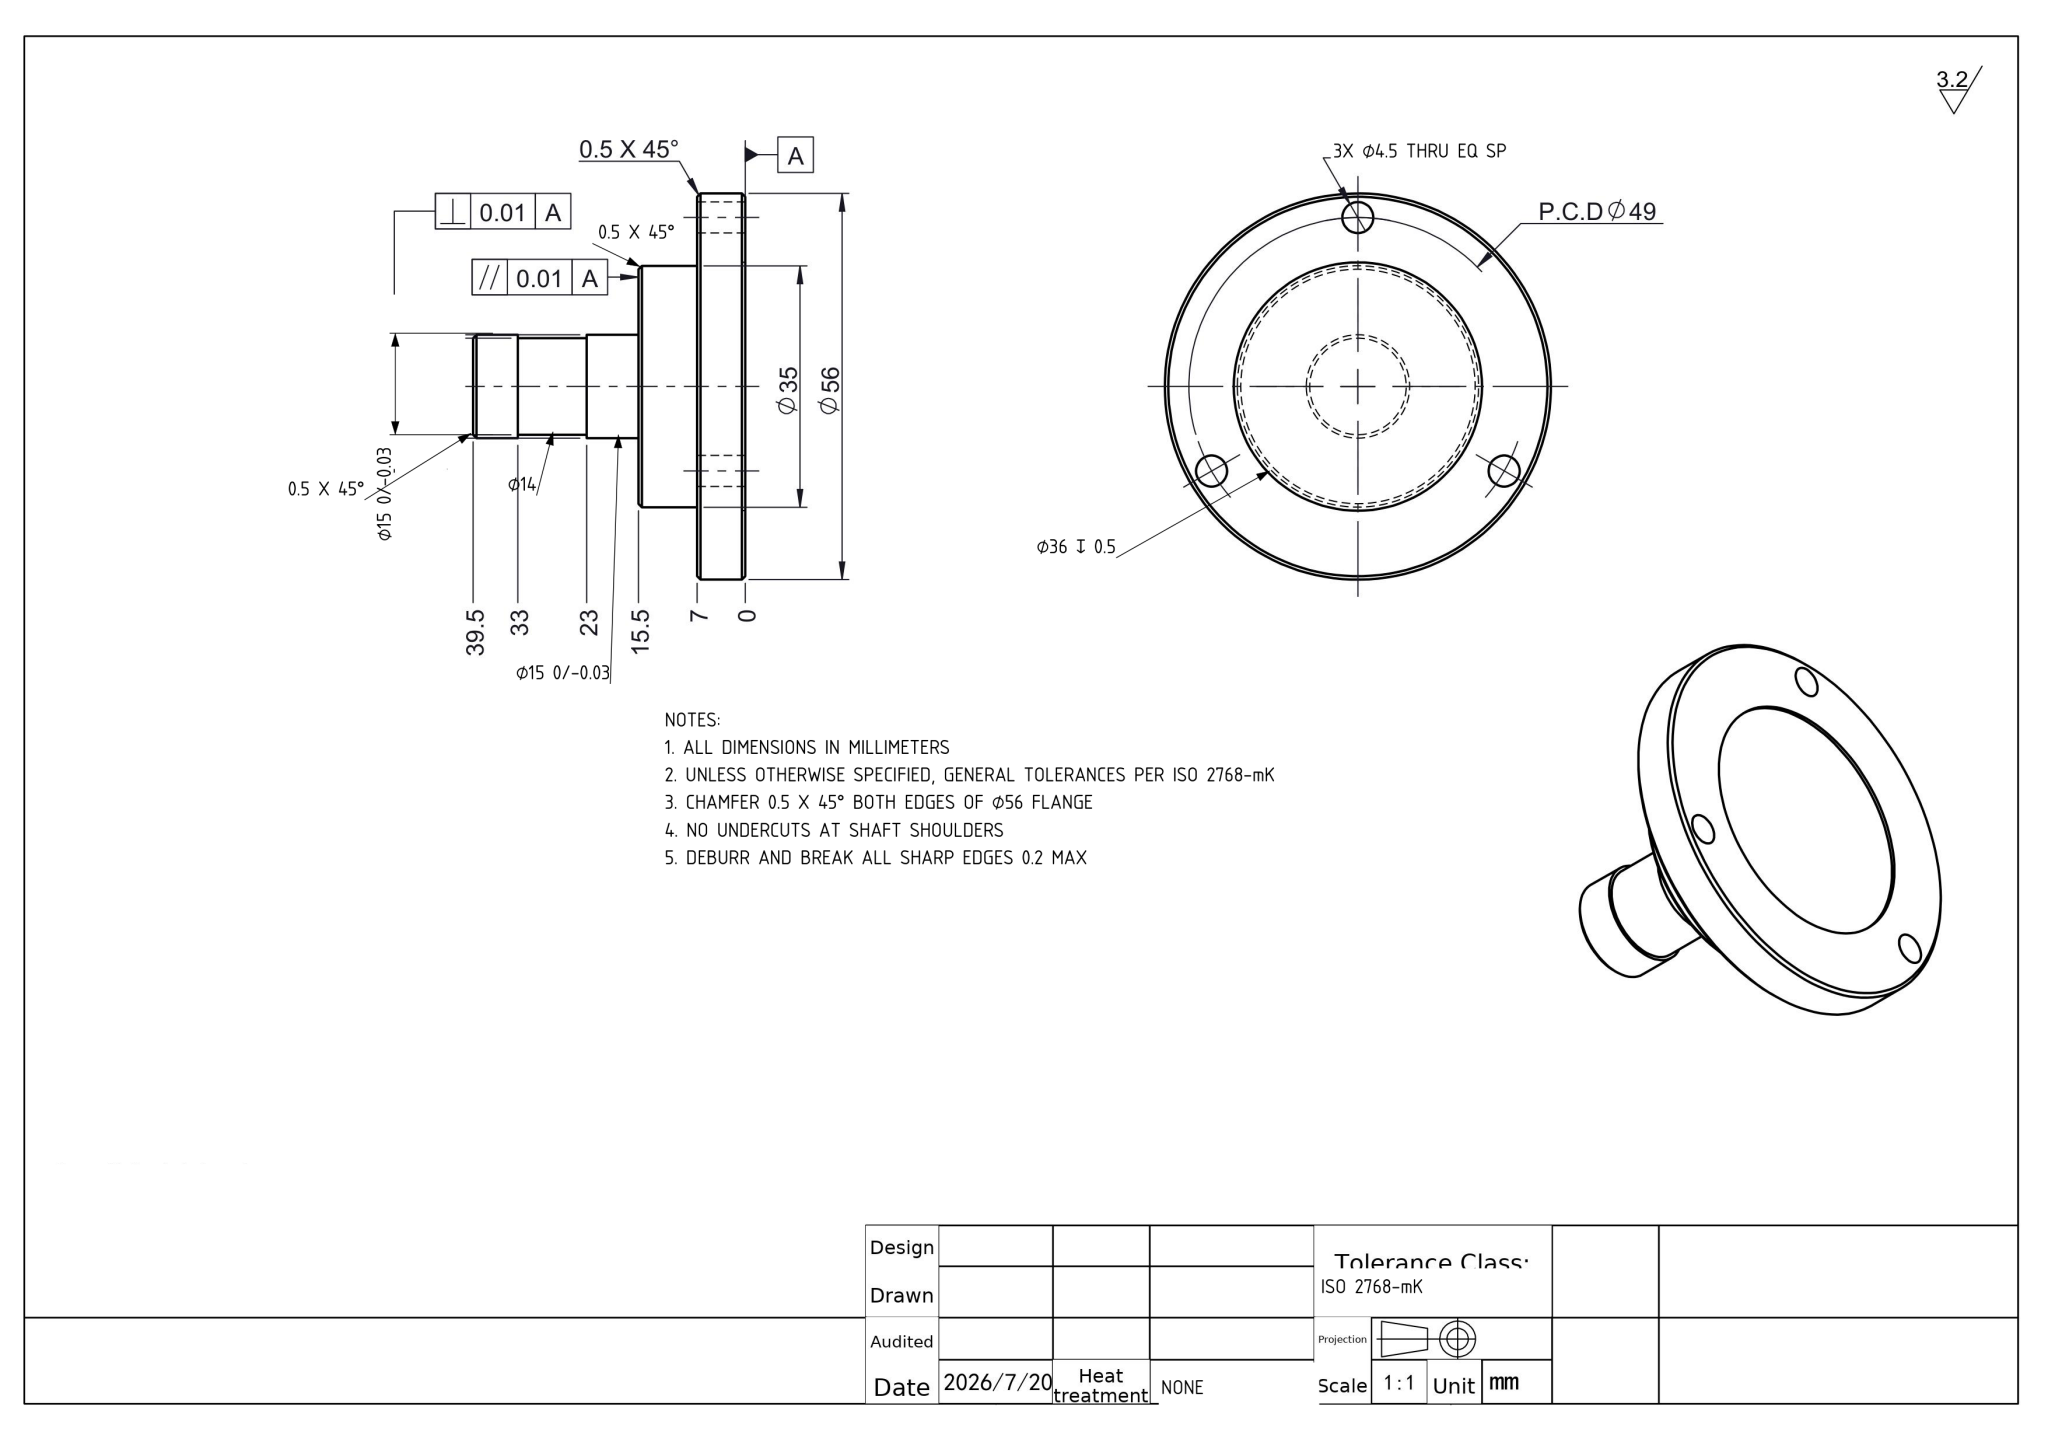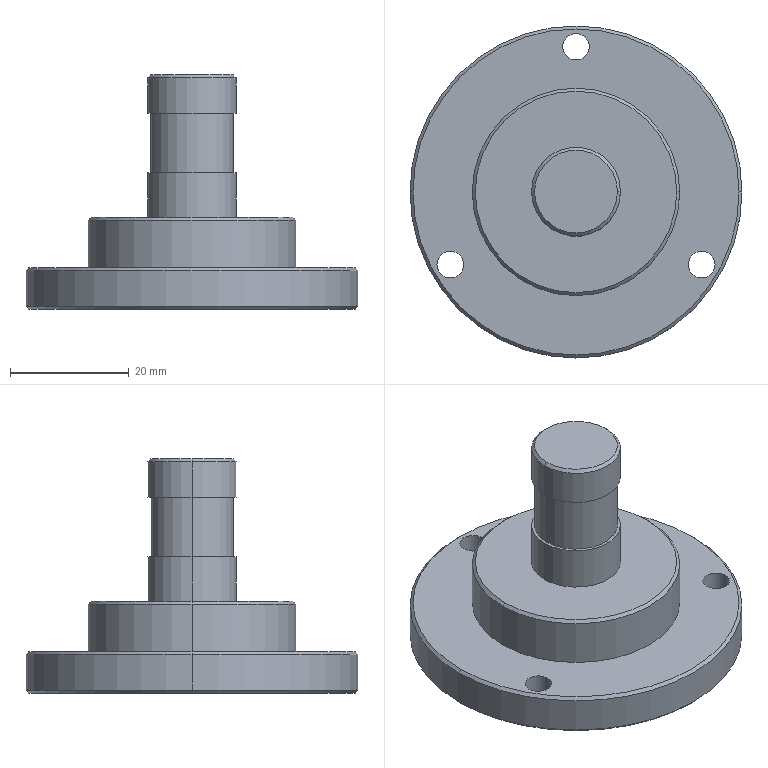Part | NX | mm | 1 solid | 33 faces | box 56 x 56 x 39.5 mm | volume 28526 mm3 | cylinder 18 | cone 8 | plane 7 | commonest cylinder face diameters 4.5 x6 15 x4 36 x2 14 x2 35 x2 56 x2
STEP:
#1=COLOUR_RGB('',0.7922,0.8196,0.9333);
#2=FILL_AREA_STYLE_COLOUR('',#1);
#3=FILL_AREA_STYLE('',(#2));
#4=SURFACE_STYLE_FILL_AREA(#3);
#5=SURFACE_SIDE_STYLE('',(#4));
#6=SURFACE_STYLE_USAGE(.BOTH.,#5);
#7=PRESENTATION_STYLE_ASSIGNMENT((#6));
#8=CARTESIAN_POINT('',(18.,0.,0.5));
#9=VERTEX_POINT('',#8);
#10=CARTESIAN_POINT('',(-18.,0.,0.5));
#11=VERTEX_POINT('',#10);
#12=CARTESIAN_POINT('',(0.,0.,0.5));
#13=DIRECTION('',(0.,0.,-1.));
#14=DIRECTION('',(-1.,0.,0.));
#15=AXIS2_PLACEMENT_3D('',#12,#13,#14);
#16=CIRCLE('',#15,18.);
#17=EDGE_CURVE('',#9,#11,#16,.T.);
#18=ORIENTED_EDGE('',*,*,#17,.F.);
#19=CARTESIAN_POINT('',(18.,0.,0.));
#20=VERTEX_POINT('',#19);
#21=CARTESIAN_POINT('',(18.,0.,0.5));
#22=DIRECTION('',(0.,0.,-1.));
#23=VECTOR('',#22,1000.);
#24=LINE('',#21,#23);
#25=EDGE_CURVE('',#9,#20,#24,.T.);
#26=ORIENTED_EDGE('',*,*,#25,.T.);
#27=CARTESIAN_POINT('',(-18.,0.,0.));
#28=VERTEX_POINT('',#27);
#29=CARTESIAN_POINT('',(0.,0.,0.));
#30=DIRECTION('',(0.,0.,-1.));
#31=DIRECTION('',(-1.,0.,0.));
#32=AXIS2_PLACEMENT_3D('',#29,#30,#31);
#33=CIRCLE('',#32,18.);
#34=EDGE_CURVE('',#20,#28,#33,.T.);
#35=ORIENTED_EDGE('',*,*,#34,.T.);
#36=CARTESIAN_POINT('',(-18.,0.,0.5));
#37=DIRECTION('',(0.,0.,-1.));
#38=VECTOR('',#37,1000.);
#39=LINE('',#36,#38);
#40=EDGE_CURVE('',#11,#28,#39,.T.);
#41=ORIENTED_EDGE('',*,*,#40,.F.);
#42=EDGE_LOOP('',(#18,#26,#35,#41));
#43=FACE_OUTER_BOUND('',#42,.T.);
#44=CARTESIAN_POINT('',(0.,0.,0.5));
#45=DIRECTION('',(0.,0.,-1.));
#46=DIRECTION('',(-1.,0.,0.));
#47=AXIS2_PLACEMENT_3D('',#44,#45,#46);
#48=CYLINDRICAL_SURFACE('',#47,18.);
#49=ADVANCED_FACE('',(#43),#48,.F.);
#50=CARTESIAN_POINT('',(7.,0.,39.5));
#51=VERTEX_POINT('',#50);
#52=CARTESIAN_POINT('',(-7.,0.,39.5));
#53=VERTEX_POINT('',#52);
#54=CARTESIAN_POINT('',(0.,0.,39.5));
#55=DIRECTION('',(0.,0.,1.));
#56=DIRECTION('',(1.,0.,0.));
#57=AXIS2_PLACEMENT_3D('',#54,#55,#56);
#58=CIRCLE('',#57,7.);
#59=EDGE_CURVE('',#51,#53,#58,.T.);
#60=ORIENTED_EDGE('',*,*,#59,.F.);
#61=CARTESIAN_POINT('',(7.5,0.,39.));
#62=VERTEX_POINT('',#61);
#63=CARTESIAN_POINT('',(7.,0.,39.5));
#64=DIRECTION('',(0.7071,0.,-0.7071));
#65=VECTOR('',#64,1000.);
#66=LINE('',#63,#65);
#67=EDGE_CURVE('',#51,#62,#66,.T.);
#68=ORIENTED_EDGE('',*,*,#67,.T.);
#69=CARTESIAN_POINT('',(-7.5,0.,39.));
#70=VERTEX_POINT('',#69);
#71=CARTESIAN_POINT('',(0.,0.,39.));
#72=DIRECTION('',(0.,0.,-1.));
#73=DIRECTION('',(1.,0.,0.));
#74=AXIS2_PLACEMENT_3D('',#71,#72,#73);
#75=CIRCLE('',#74,7.5);
#76=EDGE_CURVE('',#70,#62,#75,.T.);
#77=ORIENTED_EDGE('',*,*,#76,.F.);
#78=CARTESIAN_POINT('',(-7.,0.,39.5));
#79=DIRECTION('',(-0.7071,0.,-0.7071));
#80=VECTOR('',#79,1000.);
#81=LINE('',#78,#80);
#82=EDGE_CURVE('',#53,#70,#81,.T.);
#83=ORIENTED_EDGE('',*,*,#82,.F.);
#84=EDGE_LOOP('',(#60,#68,#77,#83));
#85=FACE_OUTER_BOUND('',#84,.T.);
#86=CARTESIAN_POINT('',(0.,0.,39.5));
#87=DIRECTION('',(0.,0.,-1.));
#88=DIRECTION('',(-1.,0.,0.));
#89=AXIS2_PLACEMENT_3D('',#86,#87,#88);
#90=CONICAL_SURFACE('',#89,7.,0.7854);
#91=ADVANCED_FACE('',(#85),#90,.T.);
#92=CARTESIAN_POINT('',(17.,0.,15.5));
#93=VERTEX_POINT('',#92);
#94=CARTESIAN_POINT('',(-17.,0.,15.5));
#95=VERTEX_POINT('',#94);
#96=CARTESIAN_POINT('',(0.,0.,15.5));
#97=DIRECTION('',(0.,0.,1.));
#98=DIRECTION('',(1.,0.,0.));
#99=AXIS2_PLACEMENT_3D('',#96,#97,#98);
#100=CIRCLE('',#99,17.);
#101=EDGE_CURVE('',#93,#95,#100,.T.);
#102=ORIENTED_EDGE('',*,*,#101,.F.);
#103=CARTESIAN_POINT('',(17.5,0.,15.));
#104=VERTEX_POINT('',#103);
#105=CARTESIAN_POINT('',(17.,0.,15.5));
#106=DIRECTION('',(0.7071,0.,-0.7071));
#107=VECTOR('',#106,1000.);
#108=LINE('',#105,#107);
#109=EDGE_CURVE('',#93,#104,#108,.T.);
#110=ORIENTED_EDGE('',*,*,#109,.T.);
#111=CARTESIAN_POINT('',(-17.5,0.,15.));
#112=VERTEX_POINT('',#111);
#113=CARTESIAN_POINT('',(0.,0.,15.));
#114=DIRECTION('',(0.,0.,-1.));
#115=DIRECTION('',(1.,0.,0.));
#116=AXIS2_PLACEMENT_3D('',#113,#114,#115);
#117=CIRCLE('',#116,17.5);
#118=EDGE_CURVE('',#112,#104,#117,.T.);
#119=ORIENTED_EDGE('',*,*,#118,.F.);
#120=CARTESIAN_POINT('',(-17.,0.,15.5));
#121=DIRECTION('',(-0.7071,0.,-0.7071));
#122=VECTOR('',#121,1000.);
#123=LINE('',#120,#122);
#124=EDGE_CURVE('',#95,#112,#123,.T.);
#125=ORIENTED_EDGE('',*,*,#124,.F.);
#126=EDGE_LOOP('',(#102,#110,#119,#125));
#127=FACE_OUTER_BOUND('',#126,.T.);
#128=CARTESIAN_POINT('',(0.,0.,15.5));
#129=DIRECTION('',(0.,0.,-1.));
#130=DIRECTION('',(-1.,0.,0.));
#131=AXIS2_PLACEMENT_3D('',#128,#129,#130);
#132=CONICAL_SURFACE('',#131,17.,0.7854);
#133=ADVANCED_FACE('',(#127),#132,.T.);
#134=CARTESIAN_POINT('',(27.5,0.,7.));
#135=VERTEX_POINT('',#134);
#136=CARTESIAN_POINT('',(-27.5,0.,7.));
#137=VERTEX_POINT('',#136);
#138=CARTESIAN_POINT('',(0.,0.,7.));
#139=DIRECTION('',(0.,0.,1.));
#140=DIRECTION('',(1.,0.,0.));
#141=AXIS2_PLACEMENT_3D('',#138,#139,#140);
#142=CIRCLE('',#141,27.5);
#143=EDGE_CURVE('',#135,#137,#142,.T.);
#144=ORIENTED_EDGE('',*,*,#143,.F.);
#145=CARTESIAN_POINT('',(28.,0.,6.5));
#146=VERTEX_POINT('',#145);
#147=CARTESIAN_POINT('',(27.5,0.,7.));
#148=DIRECTION('',(0.7071,0.,-0.7071));
#149=VECTOR('',#148,1000.);
#150=LINE('',#147,#149);
#151=EDGE_CURVE('',#135,#146,#150,.T.);
#152=ORIENTED_EDGE('',*,*,#151,.T.);
#153=CARTESIAN_POINT('',(-28.,0.,6.5));
#154=VERTEX_POINT('',#153);
#155=CARTESIAN_POINT('',(0.,0.,6.5));
#156=DIRECTION('',(0.,0.,-1.));
#157=DIRECTION('',(1.,0.,0.));
#158=AXIS2_PLACEMENT_3D('',#155,#156,#157);
#159=CIRCLE('',#158,28.);
#160=EDGE_CURVE('',#154,#146,#159,.T.);
#161=ORIENTED_EDGE('',*,*,#160,.F.);
#162=CARTESIAN_POINT('',(-27.5,0.,7.));
#163=DIRECTION('',(-0.7071,0.,-0.7071));
#164=VECTOR('',#163,1000.);
#165=LINE('',#162,#164);
#166=EDGE_CURVE('',#137,#154,#165,.T.);
#167=ORIENTED_EDGE('',*,*,#166,.F.);
#168=EDGE_LOOP('',(#144,#152,#161,#167));
#169=FACE_OUTER_BOUND('',#168,.T.);
#170=CARTESIAN_POINT('',(0.,0.,7.));
#171=DIRECTION('',(0.,0.,-1.));
#172=DIRECTION('',(-1.,0.,0.));
#173=AXIS2_PLACEMENT_3D('',#170,#171,#172);
#174=CONICAL_SURFACE('',#173,27.5,0.7854);
#175=ADVANCED_FACE('',(#169),#174,.T.);
#176=CARTESIAN_POINT('',(-27.5,0.,0.));
#177=VERTEX_POINT('',#176);
#178=CARTESIAN_POINT('',(27.5,0.,0.));
#179=VERTEX_POINT('',#178);
#180=CARTESIAN_POINT('',(0.,0.,0.));
#181=DIRECTION('',(0.,0.,-1.));
#182=DIRECTION('',(1.,0.,0.));
#183=AXIS2_PLACEMENT_3D('',#180,#181,#182);
#184=CIRCLE('',#183,27.5);
#185=EDGE_CURVE('',#177,#179,#184,.T.);
#186=ORIENTED_EDGE('',*,*,#185,.F.);
#187=CARTESIAN_POINT('',(-28.,0.,0.5));
#188=VERTEX_POINT('',#187);
#189=CARTESIAN_POINT('',(-28.,0.,0.5));
#190=DIRECTION('',(-0.7071,0.,0.7071));
#191=VECTOR('',#190,1000.);
#192=LINE('',#189,#191);
#193=EDGE_CURVE('',#177,#188,#192,.T.);
#194=ORIENTED_EDGE('',*,*,#193,.T.);
#195=CARTESIAN_POINT('',(28.,0.,0.5));
#196=VERTEX_POINT('',#195);
#197=CARTESIAN_POINT('',(0.,0.,0.5));
#198=DIRECTION('',(0.,0.,1.));
#199=DIRECTION('',(1.,0.,0.));
#200=AXIS2_PLACEMENT_3D('',#197,#198,#199);
#201=CIRCLE('',#200,28.);
#202=EDGE_CURVE('',#196,#188,#201,.T.);
#203=ORIENTED_EDGE('',*,*,#202,.F.);
#204=CARTESIAN_POINT('',(28.,0.,0.5));
#205=DIRECTION('',(0.7071,0.,0.7071));
#206=VECTOR('',#205,1000.);
#207=LINE('',#204,#206);
#208=EDGE_CURVE('',#179,#196,#207,.T.);
#209=ORIENTED_EDGE('',*,*,#208,.F.);
#210=EDGE_LOOP('',(#186,#194,#203,#209));
#211=FACE_OUTER_BOUND('',#210,.T.);
#212=CARTESIAN_POINT('',(0.,0.,0.5));
#213=DIRECTION('',(0.,0.,1.));
#214=DIRECTION('',(1.,0.,0.));
#215=AXIS2_PLACEMENT_3D('',#212,#213,#214);
#216=CONICAL_SURFACE('',#215,28.,0.7854);
#217=ADVANCED_FACE('',(#211),#216,.T.);
#218=ORIENTED_EDGE('',*,*,#76,.T.);
#219=CARTESIAN_POINT('',(7.5,0.,33.));
#220=VERTEX_POINT('',#219);
#221=CARTESIAN_POINT('',(7.5,0.,39.5));
#222=DIRECTION('',(0.,0.,-1.));
#223=VECTOR('',#222,1000.);
#224=LINE('',#221,#223);
#225=EDGE_CURVE('',#62,#220,#224,.T.);
#226=ORIENTED_EDGE('',*,*,#225,.T.);
#227=CARTESIAN_POINT('',(-7.5,0.,33.));
#228=VERTEX_POINT('',#227);
#229=CARTESIAN_POINT('',(0.,0.,33.));
#230=DIRECTION('',(0.,0.,1.));
#231=DIRECTION('',(1.,0.,0.));
#232=AXIS2_PLACEMENT_3D('',#229,#230,#231);
#233=CIRCLE('',#232,7.5);
#234=EDGE_CURVE('',#220,#228,#233,.T.);
#235=ORIENTED_EDGE('',*,*,#234,.T.);
#236=CARTESIAN_POINT('',(-7.5,0.,39.5));
#237=DIRECTION('',(0.,0.,-1.));
#238=VECTOR('',#237,1000.);
#239=LINE('',#236,#238);
#240=EDGE_CURVE('',#70,#228,#239,.T.);
#241=ORIENTED_EDGE('',*,*,#240,.F.);
#242=EDGE_LOOP('',(#218,#226,#235,#241));
#243=FACE_OUTER_BOUND('',#242,.T.);
#244=CARTESIAN_POINT('',(0.,0.,39.5));
#245=DIRECTION('',(0.,0.,-1.));
#246=DIRECTION('',(-1.,0.,0.));
#247=AXIS2_PLACEMENT_3D('',#244,#245,#246);
#248=CYLINDRICAL_SURFACE('',#247,7.5);
#249=ADVANCED_FACE('',(#243),#248,.T.);
#250=CARTESIAN_POINT('',(7.,0.,23.));
#251=VERTEX_POINT('',#250);
#252=CARTESIAN_POINT('',(-7.,0.,23.));
#253=VERTEX_POINT('',#252);
#254=CARTESIAN_POINT('',(0.,0.,23.));
#255=DIRECTION('',(0.,0.,1.));
#256=DIRECTION('',(1.,0.,0.));
#257=AXIS2_PLACEMENT_3D('',#254,#255,#256);
#258=CIRCLE('',#257,7.);
#259=EDGE_CURVE('',#251,#253,#258,.T.);
#260=ORIENTED_EDGE('',*,*,#259,.T.);
#261=CARTESIAN_POINT('',(-7.,0.,33.));
#262=VERTEX_POINT('',#261);
#263=CARTESIAN_POINT('',(-7.,0.,39.5));
#264=DIRECTION('',(0.,0.,1.));
#265=VECTOR('',#264,1000.);
#266=LINE('',#263,#265);
#267=EDGE_CURVE('',#253,#262,#266,.T.);
#268=ORIENTED_EDGE('',*,*,#267,.T.);
#269=CARTESIAN_POINT('',(7.,0.,33.));
#270=VERTEX_POINT('',#269);
#271=CARTESIAN_POINT('',(0.,0.,33.));
#272=DIRECTION('',(0.,0.,1.));
#273=DIRECTION('',(1.,0.,0.));
#274=AXIS2_PLACEMENT_3D('',#271,#272,#273);
#275=CIRCLE('',#274,7.);
#276=EDGE_CURVE('',#270,#262,#275,.T.);
#277=ORIENTED_EDGE('',*,*,#276,.F.);
#278=CARTESIAN_POINT('',(7.,0.,39.5));
#279=DIRECTION('',(0.,0.,1.));
#280=VECTOR('',#279,1000.);
#281=LINE('',#278,#280);
#282=EDGE_CURVE('',#251,#270,#281,.T.);
#283=ORIENTED_EDGE('',*,*,#282,.F.);
#284=EDGE_LOOP('',(#260,#268,#277,#283));
#285=FACE_OUTER_BOUND('',#284,.T.);
#286=CARTESIAN_POINT('',(0.,0.,39.5));
#287=DIRECTION('',(0.,0.,1.));
#288=DIRECTION('',(1.,0.,0.));
#289=AXIS2_PLACEMENT_3D('',#286,#287,#288);
#290=CYLINDRICAL_SURFACE('',#289,7.);
#291=ADVANCED_FACE('',(#285),#290,.T.);
#292=CARTESIAN_POINT('',(-2.25,24.5,7.));
#293=VERTEX_POINT('',#292);
#294=CARTESIAN_POINT('',(2.25,24.5,7.));
#295=VERTEX_POINT('',#294);
#296=CARTESIAN_POINT('',(0.,24.5,7.));
#297=DIRECTION('',(0.,0.,1.));
#298=DIRECTION('',(1.,0.,0.));
#299=AXIS2_PLACEMENT_3D('',#296,#297,#298);
#300=CIRCLE('',#299,2.25);
#301=EDGE_CURVE('',#293,#295,#300,.T.);
#302=ORIENTED_EDGE('',*,*,#301,.T.);
#303=CARTESIAN_POINT('',(2.25,24.5,-0.));
#304=VERTEX_POINT('',#303);
#305=CARTESIAN_POINT('',(2.25,24.5,0.));
#306=DIRECTION('',(0.,0.,-1.));
#307=VECTOR('',#306,1000.);
#308=LINE('',#305,#307);
#309=EDGE_CURVE('',#295,#304,#308,.T.);
#310=ORIENTED_EDGE('',*,*,#309,.T.);
#311=CARTESIAN_POINT('',(-2.25,24.5,-0.));
#312=VERTEX_POINT('',#311);
#313=CARTESIAN_POINT('',(0.,24.5,-0.));
#314=DIRECTION('',(0.,0.,-1.));
#315=DIRECTION('',(-1.,0.,0.));
#316=AXIS2_PLACEMENT_3D('',#313,#314,#315);
#317=CIRCLE('',#316,2.25);
#318=EDGE_CURVE('',#304,#312,#317,.T.);
#319=ORIENTED_EDGE('',*,*,#318,.T.);
#320=CARTESIAN_POINT('',(-2.25,24.5,0.));
#321=DIRECTION('',(0.,0.,-1.));
#322=VECTOR('',#321,1000.);
#323=LINE('',#320,#322);
#324=EDGE_CURVE('',#293,#312,#323,.T.);
#325=ORIENTED_EDGE('',*,*,#324,.F.);
#326=EDGE_LOOP('',(#302,#310,#319,#325));
#327=FACE_OUTER_BOUND('',#326,.T.);
#328=CARTESIAN_POINT('',(0.,24.5,0.));
#329=DIRECTION('',(0.,0.,-1.));
#330=DIRECTION('',(-1.,0.,0.));
#331=AXIS2_PLACEMENT_3D('',#328,#329,#330);
#332=CYLINDRICAL_SURFACE('',#331,2.25);
#333=ADVANCED_FACE('',(#327),#332,.F.);
#334=CARTESIAN_POINT('',(-23.468,-12.25,7.));
#335=VERTEX_POINT('',#334);
#336=CARTESIAN_POINT('',(-18.968,-12.25,7.));
#337=VERTEX_POINT('',#336);
#338=CARTESIAN_POINT('',(-21.218,-12.25,7.));
#339=DIRECTION('',(0.,0.,1.));
#340=DIRECTION('',(1.,0.,0.));
#341=AXIS2_PLACEMENT_3D('',#338,#339,#340);
#342=CIRCLE('',#341,2.25);
#343=EDGE_CURVE('',#335,#337,#342,.T.);
#344=ORIENTED_EDGE('',*,*,#343,.T.);
#345=CARTESIAN_POINT('',(-18.968,-12.25,-0.));
#346=VERTEX_POINT('',#345);
#347=CARTESIAN_POINT('',(-18.968,-12.25,0.));
#348=DIRECTION('',(0.,0.,-1.));
#349=VECTOR('',#348,1000.);
#350=LINE('',#347,#349);
#351=EDGE_CURVE('',#337,#346,#350,.T.);
#352=ORIENTED_EDGE('',*,*,#351,.T.);
#353=CARTESIAN_POINT('',(-23.468,-12.25,-0.));
#354=VERTEX_POINT('',#353);
#355=CARTESIAN_POINT('',(-21.218,-12.25,-0.));
#356=DIRECTION('',(0.,0.,-1.));
#357=DIRECTION('',(-1.,0.,0.));
#358=AXIS2_PLACEMENT_3D('',#355,#356,#357);
#359=CIRCLE('',#358,2.25);
#360=EDGE_CURVE('',#346,#354,#359,.T.);
#361=ORIENTED_EDGE('',*,*,#360,.T.);
#362=CARTESIAN_POINT('',(-23.468,-12.25,0.));
#363=DIRECTION('',(0.,0.,-1.));
#364=VECTOR('',#363,1000.);
#365=LINE('',#362,#364);
#366=EDGE_CURVE('',#335,#354,#365,.T.);
#367=ORIENTED_EDGE('',*,*,#366,.F.);
#368=EDGE_LOOP('',(#344,#352,#361,#367));
#369=FACE_OUTER_BOUND('',#368,.T.);
#370=CARTESIAN_POINT('',(-21.218,-12.25,0.));
#371=DIRECTION('',(0.,0.,-1.));
#372=DIRECTION('',(-1.,0.,0.));
#373=AXIS2_PLACEMENT_3D('',#370,#371,#372);
#374=CYLINDRICAL_SURFACE('',#373,2.25);
#375=ADVANCED_FACE('',(#369),#374,.F.);
#376=CARTESIAN_POINT('',(18.968,-12.25,7.));
#377=VERTEX_POINT('',#376);
#378=CARTESIAN_POINT('',(23.468,-12.25,7.));
#379=VERTEX_POINT('',#378);
#380=CARTESIAN_POINT('',(21.218,-12.25,7.));
#381=DIRECTION('',(0.,0.,1.));
#382=DIRECTION('',(1.,0.,0.));
#383=AXIS2_PLACEMENT_3D('',#380,#381,#382);
#384=CIRCLE('',#383,2.25);
#385=EDGE_CURVE('',#377,#379,#384,.T.);
#386=ORIENTED_EDGE('',*,*,#385,.T.);
#387=CARTESIAN_POINT('',(23.468,-12.25,-0.));
#388=VERTEX_POINT('',#387);
#389=CARTESIAN_POINT('',(23.468,-12.25,0.));
#390=DIRECTION('',(0.,0.,-1.));
#391=VECTOR('',#390,1000.);
#392=LINE('',#389,#391);
#393=EDGE_CURVE('',#379,#388,#392,.T.);
#394=ORIENTED_EDGE('',*,*,#393,.T.);
#395=CARTESIAN_POINT('',(18.968,-12.25,-0.));
#396=VERTEX_POINT('',#395);
#397=CARTESIAN_POINT('',(21.218,-12.25,-0.));
#398=DIRECTION('',(0.,0.,-1.));
#399=DIRECTION('',(-1.,0.,0.));
#400=AXIS2_PLACEMENT_3D('',#397,#398,#399);
#401=CIRCLE('',#400,2.25);
#402=EDGE_CURVE('',#388,#396,#401,.T.);
#403=ORIENTED_EDGE('',*,*,#402,.T.);
#404=CARTESIAN_POINT('',(18.968,-12.25,0.));
#405=DIRECTION('',(0.,0.,-1.));
#406=VECTOR('',#405,1000.);
#407=LINE('',#404,#406);
#408=EDGE_CURVE('',#377,#396,#407,.T.);
#409=ORIENTED_EDGE('',*,*,#408,.F.);
#410=EDGE_LOOP('',(#386,#394,#403,#409));
#411=FACE_OUTER_BOUND('',#410,.T.);
#412=CARTESIAN_POINT('',(21.218,-12.25,0.));
#413=DIRECTION('',(0.,0.,-1.));
#414=DIRECTION('',(-1.,0.,0.));
#415=AXIS2_PLACEMENT_3D('',#412,#413,#414);
#416=CYLINDRICAL_SURFACE('',#415,2.25);
#417=ADVANCED_FACE('',(#411),#416,.F.);
#418=ORIENTED_EDGE('',*,*,#118,.T.);
#419=CARTESIAN_POINT('',(17.5,0.,7.));
#420=VERTEX_POINT('',#419);
#421=CARTESIAN_POINT('',(17.5,0.,15.5));
#422=DIRECTION('',(0.,0.,-1.));
#423=VECTOR('',#422,1000.);
#424=LINE('',#421,#423);
#425=EDGE_CURVE('',#104,#420,#424,.T.);
#426=ORIENTED_EDGE('',*,*,#425,.T.);
#427=CARTESIAN_POINT('',(-17.5,0.,7.));
#428=VERTEX_POINT('',#427);
#429=CARTESIAN_POINT('',(0.,0.,7.));
#430=DIRECTION('',(0.,0.,1.));
#431=DIRECTION('',(1.,0.,0.));
#432=AXIS2_PLACEMENT_3D('',#429,#430,#431);
#433=CIRCLE('',#432,17.5);
#434=EDGE_CURVE('',#420,#428,#433,.T.);
#435=ORIENTED_EDGE('',*,*,#434,.T.);
#436=CARTESIAN_POINT('',(-17.5,0.,15.5));
#437=DIRECTION('',(0.,0.,-1.));
#438=VECTOR('',#437,1000.);
#439=LINE('',#436,#438);
#440=EDGE_CURVE('',#112,#428,#439,.T.);
#441=ORIENTED_EDGE('',*,*,#440,.F.);
#442=EDGE_LOOP('',(#418,#426,#435,#441));
#443=FACE_OUTER_BOUND('',#442,.T.);
#444=CARTESIAN_POINT('',(0.,0.,15.5));
#445=DIRECTION('',(0.,0.,-1.));
#446=DIRECTION('',(-1.,0.,0.));
#447=AXIS2_PLACEMENT_3D('',#444,#445,#446);
#448=CYLINDRICAL_SURFACE('',#447,17.5);
#449=ADVANCED_FACE('',(#443),#448,.T.);
#450=ORIENTED_EDGE('',*,*,#160,.T.);
#451=CARTESIAN_POINT('',(28.,0.,7.));
#452=DIRECTION('',(0.,0.,-1.));
#453=VECTOR('',#452,1000.);
#454=LINE('',#451,#453);
#455=EDGE_CURVE('',#146,#196,#454,.T.);
#456=ORIENTED_EDGE('',*,*,#455,.T.);
#457=ORIENTED_EDGE('',*,*,#202,.T.);
#458=CARTESIAN_POINT('',(-28.,0.,7.));
#459=DIRECTION('',(0.,0.,-1.));
#460=VECTOR('',#459,1000.);
#461=LINE('',#458,#460);
#462=EDGE_CURVE('',#154,#188,#461,.T.);
#463=ORIENTED_EDGE('',*,*,#462,.F.);
#464=EDGE_LOOP('',(#450,#456,#457,#463));
#465=FACE_OUTER_BOUND('',#464,.T.);
#466=CARTESIAN_POINT('',(0.,0.,7.));
#467=DIRECTION('',(0.,0.,-1.));
#468=DIRECTION('',(-1.,0.,0.));
#469=AXIS2_PLACEMENT_3D('',#466,#467,#468);
#470=CYLINDRICAL_SURFACE('',#469,28.);
#471=ADVANCED_FACE('',(#465),#470,.T.);
#472=CARTESIAN_POINT('',(7.5,0.,23.));
#473=VERTEX_POINT('',#472);
#474=CARTESIAN_POINT('',(-7.5,0.,23.));
#475=VERTEX_POINT('',#474);
#476=CARTESIAN_POINT('',(0.,0.,23.));
#477=DIRECTION('',(0.,0.,1.));
#478=DIRECTION('',(1.,0.,0.));
#479=AXIS2_PLACEMENT_3D('',#476,#477,#478);
#480=CIRCLE('',#479,7.5);
#481=EDGE_CURVE('',#473,#475,#480,.T.);
#482=ORIENTED_EDGE('',*,*,#481,.F.);
#483=CARTESIAN_POINT('',(7.5,0.,15.5));
#484=VERTEX_POINT('',#483);
#485=CARTESIAN_POINT('',(7.5,0.,39.5));
#486=DIRECTION('',(0.,0.,-1.));
#487=VECTOR('',#486,1000.);
#488=LINE('',#485,#487);
#489=EDGE_CURVE('',#473,#484,#488,.T.);
#490=ORIENTED_EDGE('',*,*,#489,.T.);
#491=CARTESIAN_POINT('',(-7.5,0.,15.5));
#492=VERTEX_POINT('',#491);
#493=CARTESIAN_POINT('',(0.,0.,15.5));
#494=DIRECTION('',(0.,0.,1.));
#495=DIRECTION('',(1.,0.,0.));
#496=AXIS2_PLACEMENT_3D('',#493,#494,#495);
#497=CIRCLE('',#496,7.5);
#498=EDGE_CURVE('',#484,#492,#497,.T.);
#499=ORIENTED_EDGE('',*,*,#498,.T.);
#500=CARTESIAN_POINT('',(-7.5,0.,39.5));
#501=DIRECTION('',(0.,0.,-1.));
#502=VECTOR('',#501,1000.);
#503=LINE('',#500,#502);
#504=EDGE_CURVE('',#475,#492,#503,.T.);
#505=ORIENTED_EDGE('',*,*,#504,.F.);
#506=EDGE_LOOP('',(#482,#490,#499,#505));
#507=FACE_OUTER_BOUND('',#506,.T.);
#508=CARTESIAN_POINT('',(0.,0.,39.5));
#509=DIRECTION('',(0.,0.,-1.));
#510=DIRECTION('',(-1.,0.,0.));
#511=AXIS2_PLACEMENT_3D('',#508,#509,#510);
#512=CYLINDRICAL_SURFACE('',#511,7.5);
#513=ADVANCED_FACE('',(#507),#512,.T.);
#514=ORIENTED_EDGE('',*,*,#489,.F.);
#515=CARTESIAN_POINT('',(0.,0.,23.));
#516=DIRECTION('',(0.,0.,1.));
#517=DIRECTION('',(1.,0.,0.));
#518=AXIS2_PLACEMENT_3D('',#515,#516,#517);
#519=CIRCLE('',#518,7.5);
#520=EDGE_CURVE('',#475,#473,#519,.T.);
#521=ORIENTED_EDGE('',*,*,#520,.F.);
#522=ORIENTED_EDGE('',*,*,#504,.T.);
#523=CARTESIAN_POINT('',(0.,0.,15.5));
#524=DIRECTION('',(0.,0.,1.));
#525=DIRECTION('',(1.,0.,0.));
#526=AXIS2_PLACEMENT_3D('',#523,#524,#525);
#527=CIRCLE('',#526,7.5);
#528=EDGE_CURVE('',#492,#484,#527,.T.);
#529=ORIENTED_EDGE('',*,*,#528,.T.);
#530=EDGE_LOOP('',(#514,#521,#522,#529));
#531=FACE_OUTER_BOUND('',#530,.T.);
#532=CARTESIAN_POINT('',(0.,0.,39.5));
#533=DIRECTION('',(0.,0.,-1.));
#534=DIRECTION('',(-1.,0.,0.));
#535=AXIS2_PLACEMENT_3D('',#532,#533,#534);
#536=CYLINDRICAL_SURFACE('',#535,7.5);
#537=ADVANCED_FACE('',(#531),#536,.T.);
#538=ORIENTED_EDGE('',*,*,#455,.F.);
#539=CARTESIAN_POINT('',(0.,0.,6.5));
#540=DIRECTION('',(0.,0.,-1.));
#541=DIRECTION('',(1.,0.,0.));
#542=AXIS2_PLACEMENT_3D('',#539,#540,#541);
#543=CIRCLE('',#542,28.);
#544=EDGE_CURVE('',#146,#154,#543,.T.);
#545=ORIENTED_EDGE('',*,*,#544,.T.);
#546=ORIENTED_EDGE('',*,*,#462,.T.);
#547=CARTESIAN_POINT('',(0.,0.,0.5));
#548=DIRECTION('',(0.,0.,1.));
#549=DIRECTION('',(1.,0.,0.));
#550=AXIS2_PLACEMENT_3D('',#547,#548,#549);
#551=CIRCLE('',#550,28.);
#552=EDGE_CURVE('',#188,#196,#551,.T.);
#553=ORIENTED_EDGE('',*,*,#552,.T.);
#554=EDGE_LOOP('',(#538,#545,#546,#553));
#555=FACE_OUTER_BOUND('',#554,.T.);
#556=CARTESIAN_POINT('',(0.,0.,7.));
#557=DIRECTION('',(0.,0.,-1.));
#558=DIRECTION('',(-1.,0.,0.));
#559=AXIS2_PLACEMENT_3D('',#556,#557,#558);
#560=CYLINDRICAL_SURFACE('',#559,28.);
#561=ADVANCED_FACE('',(#555),#560,.T.);
#562=CARTESIAN_POINT('',(0.,0.,7.));
#563=DIRECTION('',(0.,0.,1.));
#564=DIRECTION('',(1.,0.,0.));
#565=AXIS2_PLACEMENT_3D('',#562,#563,#564);
#566=CIRCLE('',#565,27.5);
#567=EDGE_CURVE('',#137,#135,#566,.T.);
#568=ORIENTED_EDGE('',*,*,#567,.T.);
#569=ORIENTED_EDGE('',*,*,#143,.T.);
#570=EDGE_LOOP('',(#568,#569));
#571=FACE_OUTER_BOUND('',#570,.T.);
#572=ORIENTED_EDGE('',*,*,#301,.F.);
#573=CARTESIAN_POINT('',(0.,24.5,7.));
#574=DIRECTION('',(0.,0.,1.));
#575=DIRECTION('',(1.,0.,0.));
#576=AXIS2_PLACEMENT_3D('',#573,#574,#575);
#577=CIRCLE('',#576,2.25);
#578=EDGE_CURVE('',#295,#293,#577,.T.);
#579=ORIENTED_EDGE('',*,*,#578,.F.);
#580=EDGE_LOOP('',(#572,#579));
#581=FACE_BOUND('',#580,.T.);
#582=ORIENTED_EDGE('',*,*,#343,.F.);
#583=CARTESIAN_POINT('',(-21.218,-12.25,7.));
#584=DIRECTION('',(0.,0.,1.));
#585=DIRECTION('',(1.,0.,0.));
#586=AXIS2_PLACEMENT_3D('',#583,#584,#585);
#587=CIRCLE('',#586,2.25);
#588=EDGE_CURVE('',#337,#335,#587,.T.);
#589=ORIENTED_EDGE('',*,*,#588,.F.);
#590=EDGE_LOOP('',(#582,#589));
#591=FACE_BOUND('',#590,.T.);
#592=ORIENTED_EDGE('',*,*,#385,.F.);
#593=CARTESIAN_POINT('',(21.218,-12.25,7.));
#594=DIRECTION('',(0.,0.,1.));
#595=DIRECTION('',(1.,0.,0.));
#596=AXIS2_PLACEMENT_3D('',#593,#594,#595);
#597=CIRCLE('',#596,2.25);
#598=EDGE_CURVE('',#379,#377,#597,.T.);
#599=ORIENTED_EDGE('',*,*,#598,.F.);
#600=EDGE_LOOP('',(#592,#599));
#601=FACE_BOUND('',#600,.T.);
#602=CARTESIAN_POINT('',(0.,0.,7.));
#603=DIRECTION('',(0.,0.,1.));
#604=DIRECTION('',(1.,0.,0.));
#605=AXIS2_PLACEMENT_3D('',#602,#603,#604);
#606=CIRCLE('',#605,17.5);
#607=EDGE_CURVE('',#428,#420,#606,.T.);
#608=ORIENTED_EDGE('',*,*,#607,.F.);
#609=ORIENTED_EDGE('',*,*,#434,.F.);
#610=EDGE_LOOP('',(#608,#609));
#611=FACE_BOUND('',#610,.T.);
#612=CARTESIAN_POINT('',(0.,0.,7.));
#613=DIRECTION('',(0.,0.,1.));
#614=DIRECTION('',(1.,0.,0.));
#615=AXIS2_PLACEMENT_3D('',#612,#613,#614);
#616=PLANE('',#615);
#617=ADVANCED_FACE('',(#571,#581,#591,#601,#611),#616,.T.);
#618=CARTESIAN_POINT('',(0.,0.,0.));
#619=DIRECTION('',(0.,0.,-1.));
#620=DIRECTION('',(-1.,0.,0.));
#621=AXIS2_PLACEMENT_3D('',#618,#619,#620);
#622=CIRCLE('',#621,18.);
#623=EDGE_CURVE('',#28,#20,#622,.T.);
#624=ORIENTED_EDGE('',*,*,#623,.F.);
#625=ORIENTED_EDGE('',*,*,#34,.F.);
#626=EDGE_LOOP('',(#624,#625));
#627=FACE_BOUND('',#626,.T.);
#628=CARTESIAN_POINT('',(0.,0.,0.));
#629=DIRECTION('',(0.,0.,-1.));
#630=DIRECTION('',(1.,0.,0.));
#631=AXIS2_PLACEMENT_3D('',#628,#629,#630);
#632=CIRCLE('',#631,27.5);
#633=EDGE_CURVE('',#179,#177,#632,.T.);
#634=ORIENTED_EDGE('',*,*,#633,.T.);
#635=ORIENTED_EDGE('',*,*,#185,.T.);
#636=EDGE_LOOP('',(#634,#635));
#637=FACE_OUTER_BOUND('',#636,.T.);
#638=CARTESIAN_POINT('',(0.,24.5,-0.));
#639=DIRECTION('',(0.,0.,-1.));
#640=DIRECTION('',(-1.,0.,0.));
#641=AXIS2_PLACEMENT_3D('',#638,#639,#640);
#642=CIRCLE('',#641,2.25);
#643=EDGE_CURVE('',#312,#304,#642,.T.);
#644=ORIENTED_EDGE('',*,*,#643,.F.);
#645=ORIENTED_EDGE('',*,*,#318,.F.);
#646=EDGE_LOOP('',(#644,#645));
#647=FACE_BOUND('',#646,.T.);
#648=CARTESIAN_POINT('',(-21.218,-12.25,-0.));
#649=DIRECTION('',(0.,0.,-1.));
#650=DIRECTION('',(-1.,0.,0.));
#651=AXIS2_PLACEMENT_3D('',#648,#649,#650);
#652=CIRCLE('',#651,2.25);
#653=EDGE_CURVE('',#354,#346,#652,.T.);
#654=ORIENTED_EDGE('',*,*,#653,.F.);
#655=ORIENTED_EDGE('',*,*,#360,.F.);
#656=EDGE_LOOP('',(#654,#655));
#657=FACE_BOUND('',#656,.T.);
#658=CARTESIAN_POINT('',(21.218,-12.25,-0.));
#659=DIRECTION('',(0.,0.,-1.));
#660=DIRECTION('',(-1.,0.,0.));
#661=AXIS2_PLACEMENT_3D('',#658,#659,#660);
#662=CIRCLE('',#661,2.25);
#663=EDGE_CURVE('',#396,#388,#662,.T.);
#664=ORIENTED_EDGE('',*,*,#663,.F.);
#665=ORIENTED_EDGE('',*,*,#402,.F.);
#666=EDGE_LOOP('',(#664,#665));
#667=FACE_BOUND('',#666,.T.);
#668=CARTESIAN_POINT('',(0.,0.,0.));
#669=DIRECTION('',(0.,0.,1.));
#670=DIRECTION('',(1.,0.,0.));
#671=AXIS2_PLACEMENT_3D('',#668,#669,#670);
#672=PLANE('',#671);
#673=ADVANCED_FACE('',(#627,#637,#647,#657,#667),#672,.F.);
#674=ORIENTED_EDGE('',*,*,#425,.F.);
#675=CARTESIAN_POINT('',(0.,0.,15.));
#676=DIRECTION('',(0.,0.,-1.));
#677=DIRECTION('',(1.,0.,0.));
#678=AXIS2_PLACEMENT_3D('',#675,#676,#677);
#679=CIRCLE('',#678,17.5);
#680=EDGE_CURVE('',#104,#112,#679,.T.);
#681=ORIENTED_EDGE('',*,*,#680,.T.);
#682=ORIENTED_EDGE('',*,*,#440,.T.);
#683=ORIENTED_EDGE('',*,*,#607,.T.);
#684=EDGE_LOOP('',(#674,#681,#682,#683));
#685=FACE_OUTER_BOUND('',#684,.T.);
#686=CARTESIAN_POINT('',(0.,0.,15.5));
#687=DIRECTION('',(0.,0.,-1.));
#688=DIRECTION('',(-1.,0.,0.));
#689=AXIS2_PLACEMENT_3D('',#686,#687,#688);
#690=CYLINDRICAL_SURFACE('',#689,17.5);
#691=ADVANCED_FACE('',(#685),#690,.T.);
#692=CARTESIAN_POINT('',(0.,0.,15.5));
#693=DIRECTION('',(0.,0.,1.));
#694=DIRECTION('',(1.,0.,0.));
#695=AXIS2_PLACEMENT_3D('',#692,#693,#694);
#696=CIRCLE('',#695,17.);
#697=EDGE_CURVE('',#95,#93,#696,.T.);
#698=ORIENTED_EDGE('',*,*,#697,.T.);
#699=ORIENTED_EDGE('',*,*,#101,.T.);
#700=EDGE_LOOP('',(#698,#699));
#701=FACE_OUTER_BOUND('',#700,.T.);
#702=ORIENTED_EDGE('',*,*,#528,.F.);
#703=ORIENTED_EDGE('',*,*,#498,.F.);
#704=EDGE_LOOP('',(#702,#703));
#705=FACE_BOUND('',#704,.T.);
#706=CARTESIAN_POINT('',(0.,0.,15.5));
#707=DIRECTION('',(0.,0.,1.));
#708=DIRECTION('',(1.,0.,0.));
#709=AXIS2_PLACEMENT_3D('',#706,#707,#708);
#710=PLANE('',#709);
#711=ADVANCED_FACE('',(#701,#705),#710,.T.);
#712=ORIENTED_EDGE('',*,*,#393,.F.);
#713=ORIENTED_EDGE('',*,*,#598,.T.);
#714=ORIENTED_EDGE('',*,*,#408,.T.);
#715=ORIENTED_EDGE('',*,*,#663,.T.);
#716=EDGE_LOOP('',(#712,#713,#714,#715));
#717=FACE_OUTER_BOUND('',#716,.T.);
#718=CARTESIAN_POINT('',(21.218,-12.25,0.));
#719=DIRECTION('',(0.,0.,-1.));
#720=DIRECTION('',(-1.,0.,0.));
#721=AXIS2_PLACEMENT_3D('',#718,#719,#720);
#722=CYLINDRICAL_SURFACE('',#721,2.25);
#723=ADVANCED_FACE('',(#717),#722,.F.);
#724=ORIENTED_EDGE('',*,*,#351,.F.);
#725=ORIENTED_EDGE('',*,*,#588,.T.);
#726=ORIENTED_EDGE('',*,*,#366,.T.);
#727=ORIENTED_EDGE('',*,*,#653,.T.);
#728=EDGE_LOOP('',(#724,#725,#726,#727));
#729=FACE_OUTER_BOUND('',#728,.T.);
#730=CARTESIAN_POINT('',(-21.218,-12.25,0.));
#731=DIRECTION('',(0.,0.,-1.));
#732=DIRECTION('',(-1.,0.,0.));
#733=AXIS2_PLACEMENT_3D('',#730,#731,#732);
#734=CYLINDRICAL_SURFACE('',#733,2.25);
#735=ADVANCED_FACE('',(#729),#734,.F.);
#736=ORIENTED_EDGE('',*,*,#309,.F.);
#737=ORIENTED_EDGE('',*,*,#578,.T.);
#738=ORIENTED_EDGE('',*,*,#324,.T.);
#739=ORIENTED_EDGE('',*,*,#643,.T.);
#740=EDGE_LOOP('',(#736,#737,#738,#739));
#741=FACE_OUTER_BOUND('',#740,.T.);
#742=CARTESIAN_POINT('',(0.,24.5,0.));
#743=DIRECTION('',(0.,0.,-1.));
#744=DIRECTION('',(-1.,0.,0.));
#745=AXIS2_PLACEMENT_3D('',#742,#743,#744);
#746=CYLINDRICAL_SURFACE('',#745,2.25);
#747=ADVANCED_FACE('',(#741),#746,.F.);
#748=ORIENTED_EDGE('',*,*,#276,.T.);
#749=CARTESIAN_POINT('',(0.,0.,33.));
#750=DIRECTION('',(0.,0.,1.));
#751=DIRECTION('',(1.,0.,0.));
#752=AXIS2_PLACEMENT_3D('',#749,#750,#751);
#753=CIRCLE('',#752,7.);
#754=EDGE_CURVE('',#262,#270,#753,.T.);
#755=ORIENTED_EDGE('',*,*,#754,.T.);
#756=EDGE_LOOP('',(#748,#755));
#757=FACE_BOUND('',#756,.T.);
#758=CARTESIAN_POINT('',(0.,0.,33.));
#759=DIRECTION('',(0.,0.,1.));
#760=DIRECTION('',(1.,0.,0.));
#761=AXIS2_PLACEMENT_3D('',#758,#759,#760);
#762=CIRCLE('',#761,7.5);
#763=EDGE_CURVE('',#228,#220,#762,.T.);
#764=ORIENTED_EDGE('',*,*,#763,.F.);
#765=ORIENTED_EDGE('',*,*,#234,.F.);
#766=EDGE_LOOP('',(#764,#765));
#767=FACE_OUTER_BOUND('',#766,.T.);
#768=CARTESIAN_POINT('',(0.,7.5,33.));
#769=DIRECTION('',(0.,0.,-1.));
#770=DIRECTION('',(-1.,0.,0.));
#771=AXIS2_PLACEMENT_3D('',#768,#769,#770);
#772=PLANE('',#771);
#773=ADVANCED_FACE('',(#757,#767),#772,.T.);
#774=ORIENTED_EDGE('',*,*,#267,.F.);
#775=CARTESIAN_POINT('',(0.,0.,23.));
#776=DIRECTION('',(0.,0.,1.));
#777=DIRECTION('',(1.,0.,0.));
#778=AXIS2_PLACEMENT_3D('',#775,#776,#777);
#779=CIRCLE('',#778,7.);
#780=EDGE_CURVE('',#253,#251,#779,.T.);
#781=ORIENTED_EDGE('',*,*,#780,.T.);
#782=ORIENTED_EDGE('',*,*,#282,.T.);
#783=ORIENTED_EDGE('',*,*,#754,.F.);
#784=EDGE_LOOP('',(#774,#781,#782,#783));
#785=FACE_OUTER_BOUND('',#784,.T.);
#786=CARTESIAN_POINT('',(0.,0.,39.5));
#787=DIRECTION('',(0.,0.,1.));
#788=DIRECTION('',(1.,0.,0.));
#789=AXIS2_PLACEMENT_3D('',#786,#787,#788);
#790=CYLINDRICAL_SURFACE('',#789,7.);
#791=ADVANCED_FACE('',(#785),#790,.T.);
#792=ORIENTED_EDGE('',*,*,#520,.T.);
#793=ORIENTED_EDGE('',*,*,#481,.T.);
#794=EDGE_LOOP('',(#792,#793));
#795=FACE_OUTER_BOUND('',#794,.T.);
#796=ORIENTED_EDGE('',*,*,#259,.F.);
#797=ORIENTED_EDGE('',*,*,#780,.F.);
#798=EDGE_LOOP('',(#796,#797));
#799=FACE_BOUND('',#798,.T.);
#800=CARTESIAN_POINT('',(0.,7.5,23.));
#801=DIRECTION('',(0.,0.,1.));
#802=DIRECTION('',(1.,0.,0.));
#803=AXIS2_PLACEMENT_3D('',#800,#801,#802);
#804=PLANE('',#803);
#805=ADVANCED_FACE('',(#795,#799),#804,.T.);
#806=CARTESIAN_POINT('',(0.,0.,39.5));
#807=DIRECTION('',(0.,0.,1.));
#808=DIRECTION('',(1.,0.,0.));
#809=AXIS2_PLACEMENT_3D('',#806,#807,#808);
#810=CIRCLE('',#809,7.);
#811=EDGE_CURVE('',#53,#51,#810,.T.);
#812=ORIENTED_EDGE('',*,*,#811,.T.);
#813=ORIENTED_EDGE('',*,*,#59,.T.);
#814=EDGE_LOOP('',(#812,#813));
#815=FACE_OUTER_BOUND('',#814,.T.);
#816=CARTESIAN_POINT('',(0.,0.,39.5));
#817=DIRECTION('',(0.,0.,1.));
#818=DIRECTION('',(1.,0.,0.));
#819=AXIS2_PLACEMENT_3D('',#816,#817,#818);
#820=PLANE('',#819);
#821=ADVANCED_FACE('',(#815),#820,.T.);
#822=ORIENTED_EDGE('',*,*,#225,.F.);
#823=CARTESIAN_POINT('',(0.,0.,39.));
#824=DIRECTION('',(0.,0.,-1.));
#825=DIRECTION('',(1.,0.,0.));
#826=AXIS2_PLACEMENT_3D('',#823,#824,#825);
#827=CIRCLE('',#826,7.5);
#828=EDGE_CURVE('',#62,#70,#827,.T.);
#829=ORIENTED_EDGE('',*,*,#828,.T.);
#830=ORIENTED_EDGE('',*,*,#240,.T.);
#831=ORIENTED_EDGE('',*,*,#763,.T.);
#832=EDGE_LOOP('',(#822,#829,#830,#831));
#833=FACE_OUTER_BOUND('',#832,.T.);
#834=CARTESIAN_POINT('',(0.,0.,39.5));
#835=DIRECTION('',(0.,0.,-1.));
#836=DIRECTION('',(-1.,0.,0.));
#837=AXIS2_PLACEMENT_3D('',#834,#835,#836);
#838=CYLINDRICAL_SURFACE('',#837,7.5);
#839=ADVANCED_FACE('',(#833),#838,.T.);
#840=ORIENTED_EDGE('',*,*,#193,.F.);
#841=ORIENTED_EDGE('',*,*,#633,.F.);
#842=ORIENTED_EDGE('',*,*,#208,.T.);
#843=ORIENTED_EDGE('',*,*,#552,.F.);
#844=EDGE_LOOP('',(#840,#841,#842,#843));
#845=FACE_OUTER_BOUND('',#844,.T.);
#846=CARTESIAN_POINT('',(0.,0.,0.5));
#847=DIRECTION('',(0.,0.,1.));
#848=DIRECTION('',(1.,0.,0.));
#849=AXIS2_PLACEMENT_3D('',#846,#847,#848);
#850=CONICAL_SURFACE('',#849,28.,0.7854);
#851=ADVANCED_FACE('',(#845),#850,.T.);
#852=ORIENTED_EDGE('',*,*,#151,.F.);
#853=ORIENTED_EDGE('',*,*,#567,.F.);
#854=ORIENTED_EDGE('',*,*,#166,.T.);
#855=ORIENTED_EDGE('',*,*,#544,.F.);
#856=EDGE_LOOP('',(#852,#853,#854,#855));
#857=FACE_OUTER_BOUND('',#856,.T.);
#858=CARTESIAN_POINT('',(0.,0.,7.));
#859=DIRECTION('',(0.,0.,-1.));
#860=DIRECTION('',(-1.,0.,0.));
#861=AXIS2_PLACEMENT_3D('',#858,#859,#860);
#862=CONICAL_SURFACE('',#861,27.5,0.7854);
#863=ADVANCED_FACE('',(#857),#862,.T.);
#864=ORIENTED_EDGE('',*,*,#109,.F.);
#865=ORIENTED_EDGE('',*,*,#697,.F.);
#866=ORIENTED_EDGE('',*,*,#124,.T.);
#867=ORIENTED_EDGE('',*,*,#680,.F.);
#868=EDGE_LOOP('',(#864,#865,#866,#867));
#869=FACE_OUTER_BOUND('',#868,.T.);
#870=CARTESIAN_POINT('',(0.,0.,15.5));
#871=DIRECTION('',(0.,0.,-1.));
#872=DIRECTION('',(-1.,0.,0.));
#873=AXIS2_PLACEMENT_3D('',#870,#871,#872);
#874=CONICAL_SURFACE('',#873,17.,0.7854);
#875=ADVANCED_FACE('',(#869),#874,.T.);
#876=ORIENTED_EDGE('',*,*,#67,.F.);
#877=ORIENTED_EDGE('',*,*,#811,.F.);
#878=ORIENTED_EDGE('',*,*,#82,.T.);
#879=ORIENTED_EDGE('',*,*,#828,.F.);
#880=EDGE_LOOP('',(#876,#877,#878,#879));
#881=FACE_OUTER_BOUND('',#880,.T.);
#882=CARTESIAN_POINT('',(0.,0.,39.5));
#883=DIRECTION('',(0.,0.,-1.));
#884=DIRECTION('',(-1.,0.,0.));
#885=AXIS2_PLACEMENT_3D('',#882,#883,#884);
#886=CONICAL_SURFACE('',#885,7.,0.7854);
#887=ADVANCED_FACE('',(#881),#886,.T.);
#888=ORIENTED_EDGE('',*,*,#25,.F.);
#889=CARTESIAN_POINT('',(0.,0.,0.5));
#890=DIRECTION('',(0.,0.,-1.));
#891=DIRECTION('',(-1.,0.,0.));
#892=AXIS2_PLACEMENT_3D('',#889,#890,#891);
#893=CIRCLE('',#892,18.);
#894=EDGE_CURVE('',#11,#9,#893,.T.);
#895=ORIENTED_EDGE('',*,*,#894,.F.);
#896=ORIENTED_EDGE('',*,*,#40,.T.);
#897=ORIENTED_EDGE('',*,*,#623,.T.);
#898=EDGE_LOOP('',(#888,#895,#896,#897));
#899=FACE_OUTER_BOUND('',#898,.T.);
#900=CARTESIAN_POINT('',(0.,0.,0.5));
#901=DIRECTION('',(0.,0.,-1.));
#902=DIRECTION('',(-1.,0.,0.));
#903=AXIS2_PLACEMENT_3D('',#900,#901,#902);
#904=CYLINDRICAL_SURFACE('',#903,18.);
#905=ADVANCED_FACE('',(#899),#904,.F.);
#906=ORIENTED_EDGE('',*,*,#894,.T.);
#907=ORIENTED_EDGE('',*,*,#17,.T.);
#908=EDGE_LOOP('',(#906,#907));
#909=FACE_OUTER_BOUND('',#908,.T.);
#910=CARTESIAN_POINT('',(0.,0.,0.5));
#911=DIRECTION('',(0.,0.,-1.));
#912=DIRECTION('',(-1.,0.,0.));
#913=AXIS2_PLACEMENT_3D('',#910,#911,#912);
#914=PLANE('',#913);
#915=ADVANCED_FACE('',(#909),#914,.T.);
#916=CLOSED_SHELL('',(#49,#91,#133,#175,#217,#249,#291,#333,#375,#417,#449,#471,#513,#537,#561,#617,#673,#691,#711,#723,#735,#747,#773,#791,#805,#821,#839,#851,#863,#875,#887,#905,#915));
#917=MANIFOLD_SOLID_BREP('',#916);
#918=STYLED_ITEM('',(#7),#917);
#919=(LENGTH_UNIT()NAMED_UNIT(*)SI_UNIT(.MILLI.,.METRE.));
#920=UNCERTAINTY_MEASURE_WITH_UNIT(LENGTH_MEASURE(0.00001),#919,'','');
#921=(NAMED_UNIT(*)PLANE_ANGLE_UNIT()SI_UNIT($,.RADIAN.));
#922=(NAMED_UNIT(*)SI_UNIT($,.STERADIAN.)SOLID_ANGLE_UNIT());
#923=(GEOMETRIC_REPRESENTATION_CONTEXT(3)GLOBAL_UNCERTAINTY_ASSIGNED_CONTEXT((#920))GLOBAL_UNIT_ASSIGNED_CONTEXT((#919,#921,#922))REPRESENTATION_CONTEXT('',''));
#924=MECHANICAL_DESIGN_GEOMETRIC_PRESENTATION_REPRESENTATION('',(#918),#923);
#925=PRESENTATION_LAYER_ASSIGNMENT('','',(#918));
#926=CARTESIAN_POINT('',(0.,0.,0.));
#927=DIRECTION('',(0.,0.,1.));
#928=DIRECTION('',(1.,0.,0.));
#929=AXIS2_PLACEMENT_3D('',#926,#927,#928);
#930=(LENGTH_UNIT()NAMED_UNIT(*)SI_UNIT(.MILLI.,.METRE.));
#931=UNCERTAINTY_MEASURE_WITH_UNIT(LENGTH_MEASURE(0.00001),#930,'','');
#932=(NAMED_UNIT(*)PLANE_ANGLE_UNIT()SI_UNIT($,.RADIAN.));
#933=(NAMED_UNIT(*)SI_UNIT($,.STERADIAN.)SOLID_ANGLE_UNIT());
#934=(GEOMETRIC_REPRESENTATION_CONTEXT(3)GLOBAL_UNCERTAINTY_ASSIGNED_CONTEXT((#931))GLOBAL_UNIT_ASSIGNED_CONTEXT((#930,#932,#933))REPRESENTATION_CONTEXT('',''));
#935=ADVANCED_BREP_SHAPE_REPRESENTATION('',(#917,#929),#934);